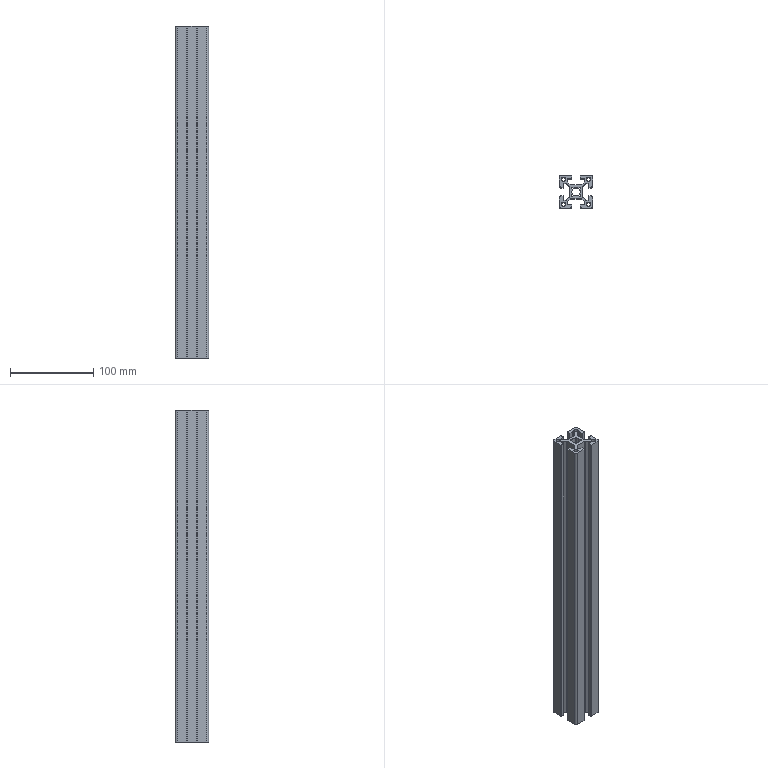Component | SolidWorks | 4040-400-1 | 1 solid | 125 faces | volume 280587 mm3 | plane 74 | cylinder 51 | commonest cylinder face diameters 2 x24 1.5 x10 5 x8 10.2 x5 4 x4